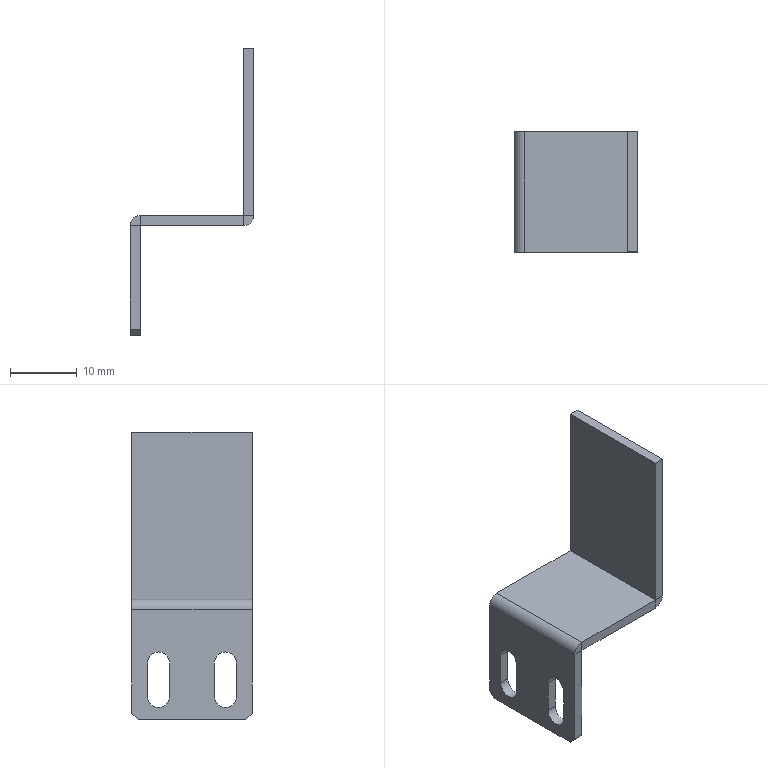Component | SolidWorks | H2020022-0439-1-1 | 1 solid | 32 faces | box 18.5 x 18 x 43 mm | volume 1526 mm3 | plane 24 | cylinder 8 | commonest cylinder face diameters 3.3 x6 3 x2 | material Stainless Steel304
STEP:
#1=COLOUR_RGB('',0.7922,0.8196,0.9333);
#2=FILL_AREA_STYLE_COLOUR('',#1);
#3=FILL_AREA_STYLE('',(#2));
#4=SURFACE_STYLE_FILL_AREA(#3);
#5=SURFACE_SIDE_STYLE('',(#4));
#6=SURFACE_STYLE_USAGE(.BOTH.,#5);
#7=PRESENTATION_STYLE_ASSIGNMENT((#6));
#8=CARTESIAN_POINT('',(1.198,-0.1393,15.794));
#9=VERTEX_POINT('',#8);
#10=CARTESIAN_POINT('',(1.198,-0.2042,15.859));
#11=VERTEX_POINT('',#10);
#12=CARTESIAN_POINT('',(1.198,-0.2042,15.794));
#13=DIRECTION('',(1.,-0.,0.));
#14=DIRECTION('',(0.,0.,-1.));
#15=AXIS2_PLACEMENT_3D('',#12,#13,#14);
#16=CIRCLE('',#15,0.06496);
#17=EDGE_CURVE('',#9,#11,#16,.T.);
#18=ORIENTED_EDGE('',*,*,#17,.T.);
#19=CARTESIAN_POINT('',(1.139,-0.2042,15.859));
#20=VERTEX_POINT('',#19);
#21=CARTESIAN_POINT('',(1.867,-0.2042,15.859));
#22=DIRECTION('',(-1.,0.,-0.));
#23=VECTOR('',#22,39.37);
#24=LINE('',#21,#23);
#25=EDGE_CURVE('',#11,#20,#24,.T.);
#26=ORIENTED_EDGE('',*,*,#25,.T.);
#27=CARTESIAN_POINT('',(1.139,-0.1393,15.794));
#28=VERTEX_POINT('',#27);
#29=CARTESIAN_POINT('',(1.139,-0.2042,15.794));
#30=DIRECTION('',(-1.,0.,-0.));
#31=DIRECTION('',(0.,-0.,1.));
#32=AXIS2_PLACEMENT_3D('',#29,#30,#31);
#33=CIRCLE('',#32,0.06496);
#34=EDGE_CURVE('',#20,#28,#33,.T.);
#35=ORIENTED_EDGE('',*,*,#34,.T.);
#36=CARTESIAN_POINT('',(1.867,-0.1393,15.794));
#37=DIRECTION('',(-1.,0.,-0.));
#38=VECTOR('',#37,39.37);
#39=LINE('',#36,#38);
#40=EDGE_CURVE('',#9,#28,#39,.T.);
#41=ORIENTED_EDGE('',*,*,#40,.F.);
#42=EDGE_LOOP('',(#18,#26,#35,#41));
#43=FACE_OUTER_BOUND('',#42,.T.);
#44=CARTESIAN_POINT('',(1.867,-0.2042,15.794));
#45=DIRECTION('',(-1.,0.,-0.));
#46=DIRECTION('',(0.,-0.,1.));
#47=AXIS2_PLACEMENT_3D('',#44,#45,#46);
#48=CYLINDRICAL_SURFACE('',#47,0.06496);
#49=ADVANCED_FACE('',(#43),#48,.F.);
#50=CARTESIAN_POINT('',(1.198,0.2544,15.794));
#51=VERTEX_POINT('',#50);
#52=CARTESIAN_POINT('',(1.198,0.1895,15.859));
#53=VERTEX_POINT('',#52);
#54=CARTESIAN_POINT('',(1.198,0.1895,15.794));
#55=DIRECTION('',(1.,-0.,0.));
#56=DIRECTION('',(0.,0.,-1.));
#57=AXIS2_PLACEMENT_3D('',#54,#55,#56);
#58=CIRCLE('',#57,0.06496);
#59=EDGE_CURVE('',#51,#53,#58,.T.);
#60=ORIENTED_EDGE('',*,*,#59,.T.);
#61=CARTESIAN_POINT('',(1.139,0.1895,15.859));
#62=VERTEX_POINT('',#61);
#63=CARTESIAN_POINT('',(1.867,0.1895,15.859));
#64=DIRECTION('',(-1.,0.,-0.));
#65=VECTOR('',#64,39.37);
#66=LINE('',#63,#65);
#67=EDGE_CURVE('',#53,#62,#66,.T.);
#68=ORIENTED_EDGE('',*,*,#67,.T.);
#69=CARTESIAN_POINT('',(1.139,0.2544,15.794));
#70=VERTEX_POINT('',#69);
#71=CARTESIAN_POINT('',(1.139,0.1895,15.794));
#72=DIRECTION('',(-1.,0.,-0.));
#73=DIRECTION('',(0.,-0.,1.));
#74=AXIS2_PLACEMENT_3D('',#71,#72,#73);
#75=CIRCLE('',#74,0.06496);
#76=EDGE_CURVE('',#62,#70,#75,.T.);
#77=ORIENTED_EDGE('',*,*,#76,.T.);
#78=CARTESIAN_POINT('',(1.867,0.2544,15.794));
#79=DIRECTION('',(-1.,0.,-0.));
#80=VECTOR('',#79,39.37);
#81=LINE('',#78,#80);
#82=EDGE_CURVE('',#51,#70,#81,.T.);
#83=ORIENTED_EDGE('',*,*,#82,.F.);
#84=EDGE_LOOP('',(#60,#68,#77,#83));
#85=FACE_OUTER_BOUND('',#84,.T.);
#86=CARTESIAN_POINT('',(1.867,0.1895,15.794));
#87=DIRECTION('',(-1.,0.,-0.));
#88=DIRECTION('',(0.,-0.,1.));
#89=AXIS2_PLACEMENT_3D('',#86,#87,#88);
#90=CYLINDRICAL_SURFACE('',#89,0.06496);
#91=ADVANCED_FACE('',(#85),#90,.F.);
#92=CARTESIAN_POINT('',(1.198,0.347,16.168));
#93=VERTEX_POINT('',#92);
#94=CARTESIAN_POINT('',(1.808,0.347,16.168));
#95=VERTEX_POINT('',#94);
#96=CARTESIAN_POINT('',(0.5288,0.347,16.168));
#97=DIRECTION('',(1.,-0.,-0.));
#98=VECTOR('',#97,39.37);
#99=LINE('',#96,#98);
#100=EDGE_CURVE('',#93,#95,#99,.T.);
#101=ORIENTED_EDGE('',*,*,#100,.T.);
#102=CARTESIAN_POINT('',(1.808,0.347,16.109));
#103=VERTEX_POINT('',#102);
#104=CARTESIAN_POINT('',(1.808,0.347,16.109));
#105=DIRECTION('',(-0.,0.,-1.));
#106=VECTOR('',#105,39.37);
#107=LINE('',#104,#106);
#108=EDGE_CURVE('',#95,#103,#107,.T.);
#109=ORIENTED_EDGE('',*,*,#108,.T.);
#110=CARTESIAN_POINT('',(1.198,0.347,16.109));
#111=VERTEX_POINT('',#110);
#112=CARTESIAN_POINT('',(0.5288,0.347,16.109));
#113=DIRECTION('',(1.,-0.,-0.));
#114=VECTOR('',#113,39.37);
#115=LINE('',#112,#114);
#116=EDGE_CURVE('',#111,#103,#115,.T.);
#117=ORIENTED_EDGE('',*,*,#116,.F.);
#118=CARTESIAN_POINT('',(1.198,0.347,16.109));
#119=DIRECTION('',(-0.,0.,-1.));
#120=VECTOR('',#119,39.37);
#121=LINE('',#118,#120);
#122=EDGE_CURVE('',#93,#111,#121,.T.);
#123=ORIENTED_EDGE('',*,*,#122,.F.);
#124=EDGE_LOOP('',(#101,#109,#117,#123));
#125=FACE_OUTER_BOUND('',#124,.T.);
#126=CARTESIAN_POINT('',(0.5288,0.347,16.109));
#127=DIRECTION('',(-0.,-1.,-0.));
#128=DIRECTION('',(1.,-0.,-0.));
#129=AXIS2_PLACEMENT_3D('',#126,#127,#128);
#130=PLANE('',#129);
#131=ADVANCED_FACE('',(#125),#130,.F.);
#132=CARTESIAN_POINT('',(1.198,-0.3617,16.168));
#133=VERTEX_POINT('',#132);
#134=CARTESIAN_POINT('',(1.808,-0.3617,16.168));
#135=VERTEX_POINT('',#134);
#136=CARTESIAN_POINT('',(0.5288,-0.3617,16.168));
#137=DIRECTION('',(1.,-0.,-0.));
#138=VECTOR('',#137,39.37);
#139=LINE('',#136,#138);
#140=EDGE_CURVE('',#133,#135,#139,.T.);
#141=ORIENTED_EDGE('',*,*,#140,.T.);
#142=CARTESIAN_POINT('',(1.808,0.347,16.168));
#143=DIRECTION('',(0.,1.,0.));
#144=VECTOR('',#143,39.37);
#145=LINE('',#142,#144);
#146=EDGE_CURVE('',#135,#95,#145,.T.);
#147=ORIENTED_EDGE('',*,*,#146,.T.);
#148=ORIENTED_EDGE('',*,*,#100,.F.);
#149=CARTESIAN_POINT('',(1.198,0.347,16.168));
#150=DIRECTION('',(0.,1.,0.));
#151=VECTOR('',#150,39.37);
#152=LINE('',#149,#151);
#153=EDGE_CURVE('',#133,#93,#152,.T.);
#154=ORIENTED_EDGE('',*,*,#153,.F.);
#155=EDGE_LOOP('',(#141,#147,#148,#154));
#156=FACE_OUTER_BOUND('',#155,.T.);
#157=CARTESIAN_POINT('',(0.5288,0.347,16.168));
#158=DIRECTION('',(-0.,0.,-1.));
#159=DIRECTION('',(-1.,0.,0.));
#160=AXIS2_PLACEMENT_3D('',#157,#158,#159);
#161=PLANE('',#160);
#162=ADVANCED_FACE('',(#156),#161,.F.);
#163=CARTESIAN_POINT('',(1.808,-0.3617,16.109));
#164=VERTEX_POINT('',#163);
#165=CARTESIAN_POINT('',(1.808,0.347,16.109));
#166=DIRECTION('',(0.,1.,0.));
#167=VECTOR('',#166,39.37);
#168=LINE('',#165,#167);
#169=EDGE_CURVE('',#164,#103,#168,.T.);
#170=ORIENTED_EDGE('',*,*,#169,.F.);
#171=CARTESIAN_POINT('',(1.198,-0.3617,16.109));
#172=VERTEX_POINT('',#171);
#173=CARTESIAN_POINT('',(0.5288,-0.3617,16.109));
#174=DIRECTION('',(1.,-0.,-0.));
#175=VECTOR('',#174,39.37);
#176=LINE('',#173,#175);
#177=EDGE_CURVE('',#172,#164,#176,.T.);
#178=ORIENTED_EDGE('',*,*,#177,.F.);
#179=CARTESIAN_POINT('',(1.198,0.347,16.109));
#180=DIRECTION('',(0.,1.,0.));
#181=VECTOR('',#180,39.37);
#182=LINE('',#179,#181);
#183=EDGE_CURVE('',#172,#111,#182,.T.);
#184=ORIENTED_EDGE('',*,*,#183,.T.);
#185=ORIENTED_EDGE('',*,*,#116,.T.);
#186=EDGE_LOOP('',(#170,#178,#184,#185));
#187=FACE_OUTER_BOUND('',#186,.T.);
#188=CARTESIAN_POINT('',(0.5288,0.347,16.109));
#189=DIRECTION('',(-0.,0.,-1.));
#190=DIRECTION('',(-1.,0.,0.));
#191=AXIS2_PLACEMENT_3D('',#188,#189,#190);
#192=PLANE('',#191);
#193=ADVANCED_FACE('',(#187),#192,.T.);
#194=CARTESIAN_POINT('',(1.808,-0.3617,16.109));
#195=DIRECTION('',(-0.,0.,-1.));
#196=VECTOR('',#195,39.37);
#197=LINE('',#194,#196);
#198=EDGE_CURVE('',#135,#164,#197,.T.);
#199=ORIENTED_EDGE('',*,*,#198,.F.);
#200=ORIENTED_EDGE('',*,*,#140,.F.);
#201=CARTESIAN_POINT('',(1.198,-0.3617,16.109));
#202=DIRECTION('',(-0.,0.,-1.));
#203=VECTOR('',#202,39.37);
#204=LINE('',#201,#203);
#205=EDGE_CURVE('',#133,#172,#204,.T.);
#206=ORIENTED_EDGE('',*,*,#205,.T.);
#207=ORIENTED_EDGE('',*,*,#177,.T.);
#208=EDGE_LOOP('',(#199,#200,#206,#207));
#209=FACE_OUTER_BOUND('',#208,.T.);
#210=CARTESIAN_POINT('',(0.5288,-0.3617,16.109));
#211=DIRECTION('',(-0.,-1.,-0.));
#212=DIRECTION('',(1.,-0.,-0.));
#213=AXIS2_PLACEMENT_3D('',#210,#211,#212);
#214=PLANE('',#213);
#215=ADVANCED_FACE('',(#209),#214,.T.);
#216=CARTESIAN_POINT('',(1.139,0.3076,15.459));
#217=VERTEX_POINT('',#216);
#218=CARTESIAN_POINT('',(1.139,-0.3223,15.459));
#219=VERTEX_POINT('',#218);
#220=CARTESIAN_POINT('',(1.139,0.347,15.459));
#221=DIRECTION('',(-0.,-1.,-0.));
#222=VECTOR('',#221,39.37);
#223=LINE('',#220,#222);
#224=EDGE_CURVE('',#217,#219,#223,.T.);
#225=ORIENTED_EDGE('',*,*,#224,.F.);
#226=CARTESIAN_POINT('',(1.198,0.3076,15.459));
#227=VERTEX_POINT('',#226);
#228=CARTESIAN_POINT('',(1.198,0.3076,15.459));
#229=DIRECTION('',(1.,-0.,0.));
#230=VECTOR('',#229,39.37);
#231=LINE('',#228,#230);
#232=EDGE_CURVE('',#217,#227,#231,.T.);
#233=ORIENTED_EDGE('',*,*,#232,.T.);
#234=CARTESIAN_POINT('',(1.198,-0.3223,15.459));
#235=VERTEX_POINT('',#234);
#236=CARTESIAN_POINT('',(1.198,0.347,15.459));
#237=DIRECTION('',(-0.,-1.,-0.));
#238=VECTOR('',#237,39.37);
#239=LINE('',#236,#238);
#240=EDGE_CURVE('',#227,#235,#239,.T.);
#241=ORIENTED_EDGE('',*,*,#240,.T.);
#242=CARTESIAN_POINT('',(1.139,-0.3223,15.459));
#243=DIRECTION('',(-1.,0.,-0.));
#244=VECTOR('',#243,39.37);
#245=LINE('',#242,#244);
#246=EDGE_CURVE('',#235,#219,#245,.T.);
#247=ORIENTED_EDGE('',*,*,#246,.T.);
#248=EDGE_LOOP('',(#225,#233,#241,#247));
#249=FACE_OUTER_BOUND('',#248,.T.);
#250=CARTESIAN_POINT('',(1.139,0.347,15.459));
#251=DIRECTION('',(0.,0.,-1.));
#252=DIRECTION('',(-1.,0.,-0.));
#253=AXIS2_PLACEMENT_3D('',#250,#251,#252);
#254=PLANE('',#253);
#255=ADVANCED_FACE('',(#249),#254,.T.);
#256=CARTESIAN_POINT('',(1.139,-0.1393,15.597));
#257=VERTEX_POINT('',#256);
#258=CARTESIAN_POINT('',(1.139,-0.1393,15.794));
#259=DIRECTION('',(-0.,0.,-1.));
#260=VECTOR('',#259,39.37);
#261=LINE('',#258,#260);
#262=EDGE_CURVE('',#28,#257,#261,.T.);
#263=ORIENTED_EDGE('',*,*,#262,.F.);
#264=ORIENTED_EDGE('',*,*,#34,.F.);
#265=CARTESIAN_POINT('',(1.139,-0.2692,15.794));
#266=VERTEX_POINT('',#265);
#267=CARTESIAN_POINT('',(1.139,-0.2042,15.794));
#268=DIRECTION('',(-1.,0.,-0.));
#269=DIRECTION('',(0.,-0.,1.));
#270=AXIS2_PLACEMENT_3D('',#267,#268,#269);
#271=CIRCLE('',#270,0.06496);
#272=EDGE_CURVE('',#266,#20,#271,.T.);
#273=ORIENTED_EDGE('',*,*,#272,.F.);
#274=CARTESIAN_POINT('',(1.139,-0.2692,15.597));
#275=VERTEX_POINT('',#274);
#276=CARTESIAN_POINT('',(1.139,-0.2692,15.794));
#277=DIRECTION('',(0.,-0.,1.));
#278=VECTOR('',#277,39.37);
#279=LINE('',#276,#278);
#280=EDGE_CURVE('',#275,#266,#279,.T.);
#281=ORIENTED_EDGE('',*,*,#280,.F.);
#282=CARTESIAN_POINT('',(1.139,-0.2042,15.597));
#283=DIRECTION('',(-1.,0.,-0.));
#284=DIRECTION('',(0.,-0.,1.));
#285=AXIS2_PLACEMENT_3D('',#282,#283,#284);
#286=CIRCLE('',#285,0.06496);
#287=EDGE_CURVE('',#257,#275,#286,.T.);
#288=ORIENTED_EDGE('',*,*,#287,.F.);
#289=EDGE_LOOP('',(#263,#264,#273,#281,#288));
#290=FACE_BOUND('',#289,.T.);
#291=CARTESIAN_POINT('',(1.139,0.2544,15.597));
#292=VERTEX_POINT('',#291);
#293=CARTESIAN_POINT('',(1.139,0.2544,15.794));
#294=DIRECTION('',(-0.,0.,-1.));
#295=VECTOR('',#294,39.37);
#296=LINE('',#293,#295);
#297=EDGE_CURVE('',#70,#292,#296,.T.);
#298=ORIENTED_EDGE('',*,*,#297,.F.);
#299=ORIENTED_EDGE('',*,*,#76,.F.);
#300=CARTESIAN_POINT('',(1.139,0.1245,15.794));
#301=VERTEX_POINT('',#300);
#302=CARTESIAN_POINT('',(1.139,0.1895,15.794));
#303=DIRECTION('',(-1.,0.,-0.));
#304=DIRECTION('',(0.,-0.,1.));
#305=AXIS2_PLACEMENT_3D('',#302,#303,#304);
#306=CIRCLE('',#305,0.06496);
#307=EDGE_CURVE('',#301,#62,#306,.T.);
#308=ORIENTED_EDGE('',*,*,#307,.F.);
#309=CARTESIAN_POINT('',(1.139,0.1245,15.597));
#310=VERTEX_POINT('',#309);
#311=CARTESIAN_POINT('',(1.139,0.1245,15.794));
#312=DIRECTION('',(0.,-0.,1.));
#313=VECTOR('',#312,39.37);
#314=LINE('',#311,#313);
#315=EDGE_CURVE('',#310,#301,#314,.T.);
#316=ORIENTED_EDGE('',*,*,#315,.F.);
#317=CARTESIAN_POINT('',(1.139,0.1895,15.597));
#318=DIRECTION('',(-1.,0.,-0.));
#319=DIRECTION('',(0.,-0.,1.));
#320=AXIS2_PLACEMENT_3D('',#317,#318,#319);
#321=CIRCLE('',#320,0.06496);
#322=EDGE_CURVE('',#292,#310,#321,.T.);
#323=ORIENTED_EDGE('',*,*,#322,.F.);
#324=EDGE_LOOP('',(#298,#299,#308,#316,#323));
#325=FACE_BOUND('',#324,.T.);
#326=CARTESIAN_POINT('',(1.139,0.347,15.498));
#327=VERTEX_POINT('',#326);
#328=CARTESIAN_POINT('',(1.139,0.347,16.109));
#329=VERTEX_POINT('',#328);
#330=CARTESIAN_POINT('',(1.139,0.347,15.459));
#331=DIRECTION('',(-0.,-0.,1.));
#332=VECTOR('',#331,39.37);
#333=LINE('',#330,#332);
#334=EDGE_CURVE('',#327,#329,#333,.T.);
#335=ORIENTED_EDGE('',*,*,#334,.F.);
#336=CARTESIAN_POINT('',(1.139,0.3076,15.459));
#337=DIRECTION('',(-0.,-0.7071,-0.7071));
#338=VECTOR('',#337,39.37);
#339=LINE('',#336,#338);
#340=EDGE_CURVE('',#327,#217,#339,.T.);
#341=ORIENTED_EDGE('',*,*,#340,.T.);
#342=ORIENTED_EDGE('',*,*,#224,.T.);
#343=CARTESIAN_POINT('',(1.139,-0.3617,15.498));
#344=VERTEX_POINT('',#343);
#345=CARTESIAN_POINT('',(1.139,-0.3617,15.498));
#346=DIRECTION('',(-0.,-0.7071,0.7071));
#347=VECTOR('',#346,39.37);
#348=LINE('',#345,#347);
#349=EDGE_CURVE('',#219,#344,#348,.T.);
#350=ORIENTED_EDGE('',*,*,#349,.T.);
#351=CARTESIAN_POINT('',(1.139,-0.3617,16.109));
#352=VERTEX_POINT('',#351);
#353=CARTESIAN_POINT('',(1.139,-0.3617,15.459));
#354=DIRECTION('',(-0.,-0.,1.));
#355=VECTOR('',#354,39.37);
#356=LINE('',#353,#355);
#357=EDGE_CURVE('',#344,#352,#356,.T.);
#358=ORIENTED_EDGE('',*,*,#357,.T.);
#359=CARTESIAN_POINT('',(1.139,0.347,16.109));
#360=DIRECTION('',(0.,1.,0.));
#361=VECTOR('',#360,39.37);
#362=LINE('',#359,#361);
#363=EDGE_CURVE('',#352,#329,#362,.T.);
#364=ORIENTED_EDGE('',*,*,#363,.T.);
#365=EDGE_LOOP('',(#335,#341,#342,#350,#358,#364));
#366=FACE_OUTER_BOUND('',#365,.T.);
#367=CARTESIAN_POINT('',(1.139,0.347,15.459));
#368=DIRECTION('',(1.,-0.,-0.));
#369=DIRECTION('',(0.,0.,-1.));
#370=AXIS2_PLACEMENT_3D('',#367,#368,#369);
#371=PLANE('',#370);
#372=ADVANCED_FACE('',(#290,#325,#366),#371,.F.);
#373=CARTESIAN_POINT('',(1.198,0.347,15.498));
#374=VERTEX_POINT('',#373);
#375=CARTESIAN_POINT('',(1.198,0.347,15.459));
#376=DIRECTION('',(-0.,-0.,1.));
#377=VECTOR('',#376,39.37);
#378=LINE('',#375,#377);
#379=EDGE_CURVE('',#374,#111,#378,.T.);
#380=ORIENTED_EDGE('',*,*,#379,.F.);
#381=CARTESIAN_POINT('',(1.139,0.347,15.498));
#382=DIRECTION('',(-1.,0.,-0.));
#383=VECTOR('',#382,39.37);
#384=LINE('',#381,#383);
#385=EDGE_CURVE('',#374,#327,#384,.T.);
#386=ORIENTED_EDGE('',*,*,#385,.T.);
#387=ORIENTED_EDGE('',*,*,#334,.T.);
#388=CARTESIAN_POINT('',(1.198,0.347,16.109));
#389=DIRECTION('',(1.,-0.,0.));
#390=VECTOR('',#389,39.37);
#391=LINE('',#388,#390);
#392=EDGE_CURVE('',#329,#111,#391,.T.);
#393=ORIENTED_EDGE('',*,*,#392,.T.);
#394=EDGE_LOOP('',(#380,#386,#387,#393));
#395=FACE_OUTER_BOUND('',#394,.T.);
#396=CARTESIAN_POINT('',(1.198,0.347,15.459));
#397=DIRECTION('',(-0.,-1.,-0.));
#398=DIRECTION('',(-0.,-0.,1.));
#399=AXIS2_PLACEMENT_3D('',#396,#397,#398);
#400=PLANE('',#399);
#401=ADVANCED_FACE('',(#395),#400,.F.);
#402=ORIENTED_EDGE('',*,*,#17,.F.);
#403=CARTESIAN_POINT('',(1.198,-0.1393,15.597));
#404=VERTEX_POINT('',#403);
#405=CARTESIAN_POINT('',(1.198,-0.1393,15.459));
#406=DIRECTION('',(-0.,-0.,1.));
#407=VECTOR('',#406,39.37);
#408=LINE('',#405,#407);
#409=EDGE_CURVE('',#404,#9,#408,.T.);
#410=ORIENTED_EDGE('',*,*,#409,.F.);
#411=CARTESIAN_POINT('',(1.198,-0.2692,15.597));
#412=VERTEX_POINT('',#411);
#413=CARTESIAN_POINT('',(1.198,-0.2042,15.597));
#414=DIRECTION('',(1.,-0.,0.));
#415=DIRECTION('',(0.,0.,-1.));
#416=AXIS2_PLACEMENT_3D('',#413,#414,#415);
#417=CIRCLE('',#416,0.06496);
#418=EDGE_CURVE('',#412,#404,#417,.T.);
#419=ORIENTED_EDGE('',*,*,#418,.F.);
#420=CARTESIAN_POINT('',(1.198,-0.2692,15.794));
#421=VERTEX_POINT('',#420);
#422=CARTESIAN_POINT('',(1.198,-0.2692,15.459));
#423=DIRECTION('',(0.,0.,-1.));
#424=VECTOR('',#423,39.37);
#425=LINE('',#422,#424);
#426=EDGE_CURVE('',#421,#412,#425,.T.);
#427=ORIENTED_EDGE('',*,*,#426,.F.);
#428=CARTESIAN_POINT('',(1.198,-0.2042,15.794));
#429=DIRECTION('',(1.,-0.,0.));
#430=DIRECTION('',(0.,0.,-1.));
#431=AXIS2_PLACEMENT_3D('',#428,#429,#430);
#432=CIRCLE('',#431,0.06496);
#433=EDGE_CURVE('',#11,#421,#432,.T.);
#434=ORIENTED_EDGE('',*,*,#433,.F.);
#435=EDGE_LOOP('',(#402,#410,#419,#427,#434));
#436=FACE_BOUND('',#435,.T.);
#437=ORIENTED_EDGE('',*,*,#59,.F.);
#438=CARTESIAN_POINT('',(1.198,0.2544,15.597));
#439=VERTEX_POINT('',#438);
#440=CARTESIAN_POINT('',(1.198,0.2544,15.459));
#441=DIRECTION('',(-0.,-0.,1.));
#442=VECTOR('',#441,39.37);
#443=LINE('',#440,#442);
#444=EDGE_CURVE('',#439,#51,#443,.T.);
#445=ORIENTED_EDGE('',*,*,#444,.F.);
#446=CARTESIAN_POINT('',(1.198,0.1245,15.597));
#447=VERTEX_POINT('',#446);
#448=CARTESIAN_POINT('',(1.198,0.1895,15.597));
#449=DIRECTION('',(1.,-0.,0.));
#450=DIRECTION('',(0.,0.,-1.));
#451=AXIS2_PLACEMENT_3D('',#448,#449,#450);
#452=CIRCLE('',#451,0.06496);
#453=EDGE_CURVE('',#447,#439,#452,.T.);
#454=ORIENTED_EDGE('',*,*,#453,.F.);
#455=CARTESIAN_POINT('',(1.198,0.1245,15.794));
#456=VERTEX_POINT('',#455);
#457=CARTESIAN_POINT('',(1.198,0.1245,15.459));
#458=DIRECTION('',(0.,0.,-1.));
#459=VECTOR('',#458,39.37);
#460=LINE('',#457,#459);
#461=EDGE_CURVE('',#456,#447,#460,.T.);
#462=ORIENTED_EDGE('',*,*,#461,.F.);
#463=CARTESIAN_POINT('',(1.198,0.1895,15.794));
#464=DIRECTION('',(1.,-0.,0.));
#465=DIRECTION('',(0.,0.,-1.));
#466=AXIS2_PLACEMENT_3D('',#463,#464,#465);
#467=CIRCLE('',#466,0.06496);
#468=EDGE_CURVE('',#53,#456,#467,.T.);
#469=ORIENTED_EDGE('',*,*,#468,.F.);
#470=EDGE_LOOP('',(#437,#445,#454,#462,#469));
#471=FACE_BOUND('',#470,.T.);
#472=ORIENTED_EDGE('',*,*,#240,.F.);
#473=CARTESIAN_POINT('',(1.198,0.3273,15.479));
#474=DIRECTION('',(0.,0.7071,0.7071));
#475=VECTOR('',#474,39.37);
#476=LINE('',#473,#475);
#477=EDGE_CURVE('',#227,#374,#476,.T.);
#478=ORIENTED_EDGE('',*,*,#477,.T.);
#479=ORIENTED_EDGE('',*,*,#379,.T.);
#480=ORIENTED_EDGE('',*,*,#183,.F.);
#481=CARTESIAN_POINT('',(1.198,-0.3617,15.498));
#482=VERTEX_POINT('',#481);
#483=CARTESIAN_POINT('',(1.198,-0.3617,15.459));
#484=DIRECTION('',(-0.,-0.,1.));
#485=VECTOR('',#484,39.37);
#486=LINE('',#483,#485);
#487=EDGE_CURVE('',#482,#172,#486,.T.);
#488=ORIENTED_EDGE('',*,*,#487,.F.);
#489=CARTESIAN_POINT('',(1.198,0.01231,15.124));
#490=DIRECTION('',(0.,0.7071,-0.7071));
#491=VECTOR('',#490,39.37);
#492=LINE('',#489,#491);
#493=EDGE_CURVE('',#482,#235,#492,.T.);
#494=ORIENTED_EDGE('',*,*,#493,.T.);
#495=EDGE_LOOP('',(#472,#478,#479,#480,#488,#494));
#496=FACE_OUTER_BOUND('',#495,.T.);
#497=CARTESIAN_POINT('',(1.198,0.347,15.459));
#498=DIRECTION('',(1.,-0.,-0.));
#499=DIRECTION('',(0.,0.,-1.));
#500=AXIS2_PLACEMENT_3D('',#497,#498,#499);
#501=PLANE('',#500);
#502=ADVANCED_FACE('',(#436,#471,#496),#501,.T.);
#503=ORIENTED_EDGE('',*,*,#357,.F.);
#504=CARTESIAN_POINT('',(1.198,-0.3617,15.498));
#505=DIRECTION('',(1.,-0.,0.));
#506=VECTOR('',#505,39.37);
#507=LINE('',#504,#506);
#508=EDGE_CURVE('',#344,#482,#507,.T.);
#509=ORIENTED_EDGE('',*,*,#508,.T.);
#510=ORIENTED_EDGE('',*,*,#487,.T.);
#511=CARTESIAN_POINT('',(1.198,-0.3617,16.109));
#512=DIRECTION('',(1.,-0.,0.));
#513=VECTOR('',#512,39.37);
#514=LINE('',#511,#513);
#515=EDGE_CURVE('',#352,#172,#514,.T.);
#516=ORIENTED_EDGE('',*,*,#515,.F.);
#517=EDGE_LOOP('',(#503,#509,#510,#516));
#518=FACE_OUTER_BOUND('',#517,.T.);
#519=CARTESIAN_POINT('',(1.198,-0.3617,15.459));
#520=DIRECTION('',(-0.,-1.,-0.));
#521=DIRECTION('',(-0.,-0.,1.));
#522=AXIS2_PLACEMENT_3D('',#519,#520,#521);
#523=PLANE('',#522);
#524=ADVANCED_FACE('',(#518),#523,.T.);
#525=CARTESIAN_POINT('',(1.198,-0.3617,16.109));
#526=DIRECTION('',(-0.,-1.,-0.));
#527=DIRECTION('',(0.,-0.,1.));
#528=AXIS2_PLACEMENT_3D('',#525,#526,#527);
#529=CIRCLE('',#528,0.05906);
#530=EDGE_CURVE('',#133,#352,#529,.T.);
#531=ORIENTED_EDGE('',*,*,#530,.F.);
#532=ORIENTED_EDGE('',*,*,#153,.T.);
#533=CARTESIAN_POINT('',(1.198,0.347,16.109));
#534=DIRECTION('',(-0.,-1.,-0.));
#535=DIRECTION('',(0.,-0.,1.));
#536=AXIS2_PLACEMENT_3D('',#533,#534,#535);
#537=CIRCLE('',#536,0.05906);
#538=EDGE_CURVE('',#93,#329,#537,.T.);
#539=ORIENTED_EDGE('',*,*,#538,.T.);
#540=ORIENTED_EDGE('',*,*,#363,.F.);
#541=EDGE_LOOP('',(#531,#532,#539,#540));
#542=FACE_OUTER_BOUND('',#541,.T.);
#543=CARTESIAN_POINT('',(1.198,-0.3617,16.109));
#544=DIRECTION('',(-0.,-1.,-0.));
#545=DIRECTION('',(0.,-0.,1.));
#546=AXIS2_PLACEMENT_3D('',#543,#544,#545);
#547=CYLINDRICAL_SURFACE('',#546,0.05906);
#548=ADVANCED_FACE('',(#542),#547,.T.);
#549=ORIENTED_EDGE('',*,*,#515,.T.);
#550=ORIENTED_EDGE('',*,*,#205,.F.);
#551=ORIENTED_EDGE('',*,*,#530,.T.);
#552=EDGE_LOOP('',(#549,#550,#551));
#553=FACE_OUTER_BOUND('',#552,.T.);
#554=CARTESIAN_POINT('',(1.198,-0.3617,16.109));
#555=DIRECTION('',(0.,1.,0.));
#556=DIRECTION('',(0.,0.,-1.));
#557=AXIS2_PLACEMENT_3D('',#554,#555,#556);
#558=PLANE('',#557);
#559=ADVANCED_FACE('',(#553),#558,.F.);
#560=ORIENTED_EDGE('',*,*,#122,.T.);
#561=ORIENTED_EDGE('',*,*,#392,.F.);
#562=ORIENTED_EDGE('',*,*,#538,.F.);
#563=EDGE_LOOP('',(#560,#561,#562));
#564=FACE_OUTER_BOUND('',#563,.T.);
#565=CARTESIAN_POINT('',(1.198,0.347,16.109));
#566=DIRECTION('',(0.,1.,0.));
#567=DIRECTION('',(0.,0.,-1.));
#568=AXIS2_PLACEMENT_3D('',#565,#566,#567);
#569=PLANE('',#568);
#570=ADVANCED_FACE('',(#564),#569,.T.);
#571=CARTESIAN_POINT('',(1.867,-0.3617,16.168));
#572=VERTEX_POINT('',#571);
#573=CARTESIAN_POINT('',(1.808,-0.3617,16.168));
#574=DIRECTION('',(0.,1.,0.));
#575=DIRECTION('',(0.,0.,-1.));
#576=AXIS2_PLACEMENT_3D('',#573,#574,#575);
#577=CIRCLE('',#576,0.05906);
#578=EDGE_CURVE('',#572,#164,#577,.T.);
#579=ORIENTED_EDGE('',*,*,#578,.F.);
#580=CARTESIAN_POINT('',(1.867,-0.3617,16.168));
#581=DIRECTION('',(1.,-0.,0.));
#582=VECTOR('',#581,39.37);
#583=LINE('',#580,#582);
#584=EDGE_CURVE('',#135,#572,#583,.T.);
#585=ORIENTED_EDGE('',*,*,#584,.F.);
#586=ORIENTED_EDGE('',*,*,#198,.T.);
#587=EDGE_LOOP('',(#579,#585,#586));
#588=FACE_OUTER_BOUND('',#587,.T.);
#589=CARTESIAN_POINT('',(1.867,-0.3617,16.168));
#590=DIRECTION('',(0.,1.,0.));
#591=DIRECTION('',(0.,0.,-1.));
#592=AXIS2_PLACEMENT_3D('',#589,#590,#591);
#593=PLANE('',#592);
#594=ADVANCED_FACE('',(#588),#593,.F.);
#595=CARTESIAN_POINT('',(1.867,0.347,16.168));
#596=VERTEX_POINT('',#595);
#597=CARTESIAN_POINT('',(1.808,0.347,16.168));
#598=DIRECTION('',(0.,1.,0.));
#599=DIRECTION('',(0.,0.,-1.));
#600=AXIS2_PLACEMENT_3D('',#597,#598,#599);
#601=CIRCLE('',#600,0.05906);
#602=EDGE_CURVE('',#596,#103,#601,.T.);
#603=ORIENTED_EDGE('',*,*,#602,.F.);
#604=CARTESIAN_POINT('',(1.867,0.347,16.168));
#605=DIRECTION('',(0.,1.,0.));
#606=VECTOR('',#605,39.37);
#607=LINE('',#604,#606);
#608=EDGE_CURVE('',#572,#596,#607,.T.);
#609=ORIENTED_EDGE('',*,*,#608,.F.);
#610=ORIENTED_EDGE('',*,*,#578,.T.);
#611=ORIENTED_EDGE('',*,*,#169,.T.);
#612=EDGE_LOOP('',(#603,#609,#610,#611));
#613=FACE_OUTER_BOUND('',#612,.T.);
#614=CARTESIAN_POINT('',(1.808,0.347,16.168));
#615=DIRECTION('',(0.,1.,0.));
#616=DIRECTION('',(0.,0.,-1.));
#617=AXIS2_PLACEMENT_3D('',#614,#615,#616);
#618=CYLINDRICAL_SURFACE('',#617,0.05906);
#619=ADVANCED_FACE('',(#613),#618,.T.);
#620=CARTESIAN_POINT('',(1.867,0.347,16.168));
#621=DIRECTION('',(1.,-0.,0.));
#622=VECTOR('',#621,39.37);
#623=LINE('',#620,#622);
#624=EDGE_CURVE('',#95,#596,#623,.T.);
#625=ORIENTED_EDGE('',*,*,#624,.T.);
#626=ORIENTED_EDGE('',*,*,#602,.T.);
#627=ORIENTED_EDGE('',*,*,#108,.F.);
#628=EDGE_LOOP('',(#625,#626,#627));
#629=FACE_OUTER_BOUND('',#628,.T.);
#630=CARTESIAN_POINT('',(1.867,0.347,16.168));
#631=DIRECTION('',(0.,1.,0.));
#632=DIRECTION('',(0.,0.,-1.));
#633=AXIS2_PLACEMENT_3D('',#630,#631,#632);
#634=PLANE('',#633);
#635=ADVANCED_FACE('',(#629),#634,.T.);
#636=CARTESIAN_POINT('',(1.867,-0.3617,17.152));
#637=VERTEX_POINT('',#636);
#638=CARTESIAN_POINT('',(1.808,-0.3617,17.152));
#639=VERTEX_POINT('',#638);
#640=CARTESIAN_POINT('',(1.867,-0.3617,17.152));
#641=DIRECTION('',(-1.,0.,-0.));
#642=VECTOR('',#641,39.37);
#643=LINE('',#640,#642);
#644=EDGE_CURVE('',#637,#639,#643,.T.);
#645=ORIENTED_EDGE('',*,*,#644,.F.);
#646=CARTESIAN_POINT('',(1.867,0.347,17.152));
#647=VERTEX_POINT('',#646);
#648=CARTESIAN_POINT('',(1.867,0.347,17.152));
#649=DIRECTION('',(-0.,-1.,-0.));
#650=VECTOR('',#649,39.37);
#651=LINE('',#648,#650);
#652=EDGE_CURVE('',#647,#637,#651,.T.);
#653=ORIENTED_EDGE('',*,*,#652,.F.);
#654=CARTESIAN_POINT('',(1.808,0.347,17.152));
#655=VERTEX_POINT('',#654);
#656=CARTESIAN_POINT('',(1.867,0.347,17.152));
#657=DIRECTION('',(-1.,0.,-0.));
#658=VECTOR('',#657,39.37);
#659=LINE('',#656,#658);
#660=EDGE_CURVE('',#647,#655,#659,.T.);
#661=ORIENTED_EDGE('',*,*,#660,.T.);
#662=CARTESIAN_POINT('',(1.808,0.347,17.152));
#663=DIRECTION('',(-0.,-1.,-0.));
#664=VECTOR('',#663,39.37);
#665=LINE('',#662,#664);
#666=EDGE_CURVE('',#655,#639,#665,.T.);
#667=ORIENTED_EDGE('',*,*,#666,.T.);
#668=EDGE_LOOP('',(#645,#653,#661,#667));
#669=FACE_OUTER_BOUND('',#668,.T.);
#670=CARTESIAN_POINT('',(1.867,0.347,17.152));
#671=DIRECTION('',(-0.,-0.,1.));
#672=DIRECTION('',(0.,1.,0.));
#673=AXIS2_PLACEMENT_3D('',#670,#671,#672);
#674=PLANE('',#673);
#675=ADVANCED_FACE('',(#669),#674,.T.);
#676=ORIENTED_EDGE('',*,*,#146,.F.);
#677=CARTESIAN_POINT('',(1.808,-0.3617,14.868));
#678=DIRECTION('',(-0.,-0.,1.));
#679=VECTOR('',#678,39.37);
#680=LINE('',#677,#679);
#681=EDGE_CURVE('',#135,#639,#680,.T.);
#682=ORIENTED_EDGE('',*,*,#681,.T.);
#683=ORIENTED_EDGE('',*,*,#666,.F.);
#684=CARTESIAN_POINT('',(1.808,0.347,14.868));
#685=DIRECTION('',(-0.,-0.,1.));
#686=VECTOR('',#685,39.37);
#687=LINE('',#684,#686);
#688=EDGE_CURVE('',#95,#655,#687,.T.);
#689=ORIENTED_EDGE('',*,*,#688,.F.);
#690=EDGE_LOOP('',(#676,#682,#683,#689));
#691=FACE_OUTER_BOUND('',#690,.T.);
#692=CARTESIAN_POINT('',(1.808,0.347,14.868));
#693=DIRECTION('',(1.,-0.,0.));
#694=DIRECTION('',(0.,0.,-1.));
#695=AXIS2_PLACEMENT_3D('',#692,#693,#694);
#696=PLANE('',#695);
#697=ADVANCED_FACE('',(#691),#696,.F.);
#698=ORIENTED_EDGE('',*,*,#681,.F.);
#699=ORIENTED_EDGE('',*,*,#584,.T.);
#700=CARTESIAN_POINT('',(1.867,-0.3617,14.868));
#701=DIRECTION('',(-0.,-0.,1.));
#702=VECTOR('',#701,39.37);
#703=LINE('',#700,#702);
#704=EDGE_CURVE('',#572,#637,#703,.T.);
#705=ORIENTED_EDGE('',*,*,#704,.T.);
#706=ORIENTED_EDGE('',*,*,#644,.T.);
#707=EDGE_LOOP('',(#698,#699,#705,#706));
#708=FACE_OUTER_BOUND('',#707,.T.);
#709=CARTESIAN_POINT('',(1.867,-0.3617,14.868));
#710=DIRECTION('',(-0.,-1.,-0.));
#711=DIRECTION('',(-0.,-0.,1.));
#712=AXIS2_PLACEMENT_3D('',#709,#710,#711);
#713=PLANE('',#712);
#714=ADVANCED_FACE('',(#708),#713,.T.);
#715=ORIENTED_EDGE('',*,*,#704,.F.);
#716=ORIENTED_EDGE('',*,*,#608,.T.);
#717=CARTESIAN_POINT('',(1.867,0.347,14.868));
#718=DIRECTION('',(-0.,-0.,1.));
#719=VECTOR('',#718,39.37);
#720=LINE('',#717,#719);
#721=EDGE_CURVE('',#596,#647,#720,.T.);
#722=ORIENTED_EDGE('',*,*,#721,.T.);
#723=ORIENTED_EDGE('',*,*,#652,.T.);
#724=EDGE_LOOP('',(#715,#716,#722,#723));
#725=FACE_OUTER_BOUND('',#724,.T.);
#726=CARTESIAN_POINT('',(1.867,0.347,14.868));
#727=DIRECTION('',(1.,-0.,0.));
#728=DIRECTION('',(0.,0.,-1.));
#729=AXIS2_PLACEMENT_3D('',#726,#727,#728);
#730=PLANE('',#729);
#731=ADVANCED_FACE('',(#725),#730,.T.);
#732=ORIENTED_EDGE('',*,*,#624,.F.);
#733=ORIENTED_EDGE('',*,*,#688,.T.);
#734=ORIENTED_EDGE('',*,*,#660,.F.);
#735=ORIENTED_EDGE('',*,*,#721,.F.);
#736=EDGE_LOOP('',(#732,#733,#734,#735));
#737=FACE_OUTER_BOUND('',#736,.T.);
#738=CARTESIAN_POINT('',(1.867,0.347,14.868));
#739=DIRECTION('',(-0.,-1.,-0.));
#740=DIRECTION('',(-0.,-0.,1.));
#741=AXIS2_PLACEMENT_3D('',#738,#739,#740);
#742=PLANE('',#741);
#743=ADVANCED_FACE('',(#737),#742,.F.);
#744=ORIENTED_EDGE('',*,*,#67,.F.);
#745=ORIENTED_EDGE('',*,*,#468,.T.);
#746=CARTESIAN_POINT('',(1.867,0.1245,15.794));
#747=DIRECTION('',(-1.,0.,-0.));
#748=VECTOR('',#747,39.37);
#749=LINE('',#746,#748);
#750=EDGE_CURVE('',#456,#301,#749,.T.);
#751=ORIENTED_EDGE('',*,*,#750,.T.);
#752=ORIENTED_EDGE('',*,*,#307,.T.);
#753=EDGE_LOOP('',(#744,#745,#751,#752));
#754=FACE_OUTER_BOUND('',#753,.T.);
#755=CARTESIAN_POINT('',(1.867,0.1895,15.794));
#756=DIRECTION('',(-1.,0.,-0.));
#757=DIRECTION('',(0.,-0.,1.));
#758=AXIS2_PLACEMENT_3D('',#755,#756,#757);
#759=CYLINDRICAL_SURFACE('',#758,0.06496);
#760=ADVANCED_FACE('',(#754),#759,.F.);
#761=ORIENTED_EDGE('',*,*,#461,.T.);
#762=CARTESIAN_POINT('',(1.867,0.1245,15.597));
#763=DIRECTION('',(-1.,0.,-0.));
#764=VECTOR('',#763,39.37);
#765=LINE('',#762,#764);
#766=EDGE_CURVE('',#447,#310,#765,.T.);
#767=ORIENTED_EDGE('',*,*,#766,.T.);
#768=ORIENTED_EDGE('',*,*,#315,.T.);
#769=ORIENTED_EDGE('',*,*,#750,.F.);
#770=EDGE_LOOP('',(#761,#767,#768,#769));
#771=FACE_OUTER_BOUND('',#770,.T.);
#772=CARTESIAN_POINT('',(1.867,0.1245,15.794));
#773=DIRECTION('',(-0.,-1.,-0.));
#774=DIRECTION('',(-0.,-0.,1.));
#775=AXIS2_PLACEMENT_3D('',#772,#773,#774);
#776=PLANE('',#775);
#777=ADVANCED_FACE('',(#771),#776,.F.);
#778=ORIENTED_EDGE('',*,*,#453,.T.);
#779=CARTESIAN_POINT('',(1.867,0.2544,15.597));
#780=DIRECTION('',(-1.,0.,-0.));
#781=VECTOR('',#780,39.37);
#782=LINE('',#779,#781);
#783=EDGE_CURVE('',#439,#292,#782,.T.);
#784=ORIENTED_EDGE('',*,*,#783,.T.);
#785=ORIENTED_EDGE('',*,*,#322,.T.);
#786=ORIENTED_EDGE('',*,*,#766,.F.);
#787=EDGE_LOOP('',(#778,#784,#785,#786));
#788=FACE_OUTER_BOUND('',#787,.T.);
#789=CARTESIAN_POINT('',(1.867,0.1895,15.597));
#790=DIRECTION('',(-1.,0.,-0.));
#791=DIRECTION('',(0.,-0.,1.));
#792=AXIS2_PLACEMENT_3D('',#789,#790,#791);
#793=CYLINDRICAL_SURFACE('',#792,0.06496);
#794=ADVANCED_FACE('',(#788),#793,.F.);
#795=ORIENTED_EDGE('',*,*,#444,.T.);
#796=ORIENTED_EDGE('',*,*,#82,.T.);
#797=ORIENTED_EDGE('',*,*,#297,.T.);
#798=ORIENTED_EDGE('',*,*,#783,.F.);
#799=EDGE_LOOP('',(#795,#796,#797,#798));
#800=FACE_OUTER_BOUND('',#799,.T.);
#801=CARTESIAN_POINT('',(1.867,0.2544,15.794));
#802=DIRECTION('',(0.,1.,0.));
#803=DIRECTION('',(0.,0.,-1.));
#804=AXIS2_PLACEMENT_3D('',#801,#802,#803);
#805=PLANE('',#804);
#806=ADVANCED_FACE('',(#800),#805,.F.);
#807=ORIENTED_EDGE('',*,*,#25,.F.);
#808=ORIENTED_EDGE('',*,*,#433,.T.);
#809=CARTESIAN_POINT('',(1.867,-0.2692,15.794));
#810=DIRECTION('',(-1.,0.,-0.));
#811=VECTOR('',#810,39.37);
#812=LINE('',#809,#811);
#813=EDGE_CURVE('',#421,#266,#812,.T.);
#814=ORIENTED_EDGE('',*,*,#813,.T.);
#815=ORIENTED_EDGE('',*,*,#272,.T.);
#816=EDGE_LOOP('',(#807,#808,#814,#815));
#817=FACE_OUTER_BOUND('',#816,.T.);
#818=CARTESIAN_POINT('',(1.867,-0.2042,15.794));
#819=DIRECTION('',(-1.,0.,-0.));
#820=DIRECTION('',(0.,-0.,1.));
#821=AXIS2_PLACEMENT_3D('',#818,#819,#820);
#822=CYLINDRICAL_SURFACE('',#821,0.06496);
#823=ADVANCED_FACE('',(#817),#822,.F.);
#824=ORIENTED_EDGE('',*,*,#426,.T.);
#825=CARTESIAN_POINT('',(1.867,-0.2692,15.597));
#826=DIRECTION('',(-1.,0.,-0.));
#827=VECTOR('',#826,39.37);
#828=LINE('',#825,#827);
#829=EDGE_CURVE('',#412,#275,#828,.T.);
#830=ORIENTED_EDGE('',*,*,#829,.T.);
#831=ORIENTED_EDGE('',*,*,#280,.T.);
#832=ORIENTED_EDGE('',*,*,#813,.F.);
#833=EDGE_LOOP('',(#824,#830,#831,#832));
#834=FACE_OUTER_BOUND('',#833,.T.);
#835=CARTESIAN_POINT('',(1.867,-0.2692,15.794));
#836=DIRECTION('',(-0.,-1.,-0.));
#837=DIRECTION('',(-0.,-0.,1.));
#838=AXIS2_PLACEMENT_3D('',#835,#836,#837);
#839=PLANE('',#838);
#840=ADVANCED_FACE('',(#834),#839,.F.);
#841=ORIENTED_EDGE('',*,*,#418,.T.);
#842=CARTESIAN_POINT('',(1.867,-0.1393,15.597));
#843=DIRECTION('',(-1.,0.,-0.));
#844=VECTOR('',#843,39.37);
#845=LINE('',#842,#844);
#846=EDGE_CURVE('',#404,#257,#845,.T.);
#847=ORIENTED_EDGE('',*,*,#846,.T.);
#848=ORIENTED_EDGE('',*,*,#287,.T.);
#849=ORIENTED_EDGE('',*,*,#829,.F.);
#850=EDGE_LOOP('',(#841,#847,#848,#849));
#851=FACE_OUTER_BOUND('',#850,.T.);
#852=CARTESIAN_POINT('',(1.867,-0.2042,15.597));
#853=DIRECTION('',(-1.,0.,-0.));
#854=DIRECTION('',(0.,-0.,1.));
#855=AXIS2_PLACEMENT_3D('',#852,#853,#854);
#856=CYLINDRICAL_SURFACE('',#855,0.06496);
#857=ADVANCED_FACE('',(#851),#856,.F.);
#858=ORIENTED_EDGE('',*,*,#409,.T.);
#859=ORIENTED_EDGE('',*,*,#40,.T.);
#860=ORIENTED_EDGE('',*,*,#262,.T.);
#861=ORIENTED_EDGE('',*,*,#846,.F.);
#862=EDGE_LOOP('',(#858,#859,#860,#861));
#863=FACE_OUTER_BOUND('',#862,.T.);
#864=CARTESIAN_POINT('',(1.867,-0.1393,15.794));
#865=DIRECTION('',(0.,1.,0.));
#866=DIRECTION('',(0.,0.,-1.));
#867=AXIS2_PLACEMENT_3D('',#864,#865,#866);
#868=PLANE('',#867);
#869=ADVANCED_FACE('',(#863),#868,.F.);
#870=ORIENTED_EDGE('',*,*,#340,.F.);
#871=ORIENTED_EDGE('',*,*,#385,.F.);
#872=ORIENTED_EDGE('',*,*,#477,.F.);
#873=ORIENTED_EDGE('',*,*,#232,.F.);
#874=EDGE_LOOP('',(#870,#871,#872,#873));
#875=FACE_OUTER_BOUND('',#874,.T.);
#876=CARTESIAN_POINT('',(1.139,0.3076,15.459));
#877=DIRECTION('',(0.,0.7071,-0.7071));
#878=DIRECTION('',(-1.,0.,-0.));
#879=AXIS2_PLACEMENT_3D('',#876,#877,#878);
#880=PLANE('',#879);
#881=ADVANCED_FACE('',(#875),#880,.T.);
#882=ORIENTED_EDGE('',*,*,#349,.F.);
#883=ORIENTED_EDGE('',*,*,#246,.F.);
#884=ORIENTED_EDGE('',*,*,#493,.F.);
#885=ORIENTED_EDGE('',*,*,#508,.F.);
#886=EDGE_LOOP('',(#882,#883,#884,#885));
#887=FACE_OUTER_BOUND('',#886,.T.);
#888=CARTESIAN_POINT('',(1.198,-0.3617,15.498));
#889=DIRECTION('',(0.,0.7071,0.7071));
#890=DIRECTION('',(1.,-0.,0.));
#891=AXIS2_PLACEMENT_3D('',#888,#889,#890);
#892=PLANE('',#891);
#893=ADVANCED_FACE('',(#887),#892,.F.);
#894=CLOSED_SHELL('',(#49,#91,#131,#162,#193,#215,#255,#372,#401,#502,#524,#548,#559,#570,#594,#619,#635,#675,#697,#714,#731,#743,#760,#777,#794,#806,#823,#840,#857,#869,#881,#893));
#895=MANIFOLD_SOLID_BREP('',#894);
#896=STYLED_ITEM('',(#7),#895);
#897=(LENGTH_UNIT()NAMED_UNIT(*)SI_UNIT($,.METRE.));
#898=LENGTH_MEASURE_WITH_UNIT(LENGTH_MEASURE(0.0254),#897);
#899=DIMENSIONAL_EXPONENTS(1.,0.,0.,0.,0.,0.,0.);
#900=(CONVERSION_BASED_UNIT('',#898)LENGTH_UNIT()NAMED_UNIT(#899));
#901=UNCERTAINTY_MEASURE_WITH_UNIT(LENGTH_MEASURE(0.00001),#900,'','');
#902=(NAMED_UNIT(*)PLANE_ANGLE_UNIT()SI_UNIT($,.RADIAN.));
#903=(NAMED_UNIT(*)SI_UNIT($,.STERADIAN.)SOLID_ANGLE_UNIT());
#904=(GEOMETRIC_REPRESENTATION_CONTEXT(3)GLOBAL_UNCERTAINTY_ASSIGNED_CONTEXT((#901))GLOBAL_UNIT_ASSIGNED_CONTEXT((#900,#902,#903))REPRESENTATION_CONTEXT('',''));
#905=MECHANICAL_DESIGN_GEOMETRIC_PRESENTATION_REPRESENTATION('',(#896),#904);
#906=PRESENTATION_LAYER_ASSIGNMENT('','',(#896));
#907=CARTESIAN_POINT('',(0.,0.,0.));
#908=DIRECTION('',(0.,0.,1.));
#909=DIRECTION('',(1.,0.,0.));
#910=AXIS2_PLACEMENT_3D('',#907,#908,#909);
#911=(LENGTH_UNIT()NAMED_UNIT(*)SI_UNIT($,.METRE.));
#912=LENGTH_MEASURE_WITH_UNIT(LENGTH_MEASURE(0.0254),#911);
#913=DIMENSIONAL_EXPONENTS(1.,0.,0.,0.,0.,0.,0.);
#914=(CONVERSION_BASED_UNIT('',#912)LENGTH_UNIT()NAMED_UNIT(#913));
#915=UNCERTAINTY_MEASURE_WITH_UNIT(LENGTH_MEASURE(0.00001),#914,'','');
#916=(NAMED_UNIT(*)PLANE_ANGLE_UNIT()SI_UNIT($,.RADIAN.));
#917=(NAMED_UNIT(*)SI_UNIT($,.STERADIAN.)SOLID_ANGLE_UNIT());
#918=(GEOMETRIC_REPRESENTATION_CONTEXT(3)GLOBAL_UNCERTAINTY_ASSIGNED_CONTEXT((#915))GLOBAL_UNIT_ASSIGNED_CONTEXT((#914,#916,#917))REPRESENTATION_CONTEXT('',''));
#919=ADVANCED_BREP_SHAPE_REPRESENTATION('',(#895,#910),#918);